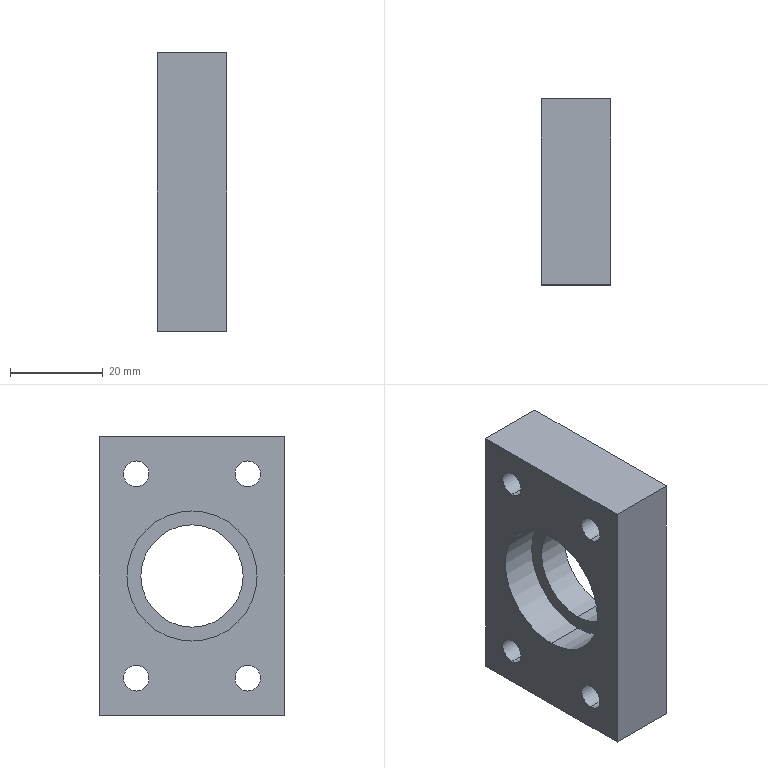Component | SolidWorks | ElectricalBoxAssembly2-1_BearingHousing-1 | 1 solid | 31 faces | box 15 x 40 x 60 mm | volume 26190 mm3 | cylinder 20 | plane 11 | commonest cylinder face diameters 9 x8 5.5 x8 22 x2 28 x2
build123d program:
from build123d import *

# Parameters (mm, degrees)
SKETCH1_W                                       = 60
SKETCH1_H                                       = 40
BOSS_EXTRUDE1_DEPTH                             = 7.5
SKETCH2_R                                       = 14
CUT_EXTRUDE1_DEPTH                              = 8
SKETCH6_R                                       = 11
CUT_EXTRUDE3_DEPTH                              = 37.932
M5_HEX_SOCKET_HEAD_CAP_SCREW_CBORE1_D           = 5.5
M5_HEX_SOCKET_HEAD_CAP_SCREW_CBORE1_CBORE_D     = 9
M5_HEX_SOCKET_HEAD_CAP_SCREW_CBORE1_CBORE_DEPTH = 5


with BuildPart() as part:
    # Sketch1 → Boss-Extrude1 (new, symmetric)
    with BuildSketch(Plane.XY):
        Rectangle(SKETCH1_W, SKETCH1_H)
    extrude(amount=BOSS_EXTRUDE1_DEPTH, both=True)

    # Sketch2 → Cut-Extrude1 (cut)
    with BuildSketch(Plane.XY.offset(7.5)):
        Circle(SKETCH2_R)
    extrude(amount=-CUT_EXTRUDE1_DEPTH, mode=Mode.SUBTRACT)

    # Sketch6 → Cut-Extrude3 (cut, through all)
    with BuildSketch(Plane.XY.offset(-0.5)):
        Circle(SKETCH6_R)
    extrude(amount=-CUT_EXTRUDE3_DEPTH, mode=Mode.SUBTRACT)

    # M5 Hex Socket Head Cap Screw CBORE1 (through all)
    with Locations(Plane(origin=(0, 0, -7.5), x_dir=(-1, 0, 0), z_dir=(0, 0, -1))):
        with Locations((-22, 12), (22, 12), (22, -12), (-22, -12)):
            CounterBoreHole(M5_HEX_SOCKET_HEAD_CAP_SCREW_CBORE1_D / 2, M5_HEX_SOCKET_HEAD_CAP_SCREW_CBORE1_CBORE_D / 2, M5_HEX_SOCKET_HEAD_CAP_SCREW_CBORE1_CBORE_DEPTH)


solid = part.part

# Placed as in the assembly
solid = solid.moved(Location((776.468, 214.666, 1676.399), (0, -90, 0)))
STEP:
#1=COLOUR_RGB('',0.7922,0.8196,0.9333);
#2=FILL_AREA_STYLE_COLOUR('',#1);
#3=FILL_AREA_STYLE('',(#2));
#4=SURFACE_STYLE_FILL_AREA(#3);
#5=SURFACE_SIDE_STYLE('',(#4));
#6=SURFACE_STYLE_USAGE(.BOTH.,#5);
#7=PRESENTATION_STYLE_ASSIGNMENT((#6));
#8=CARTESIAN_POINT('',(30.668,7.979,64.957));
#9=VERTEX_POINT('',#8);
#10=CARTESIAN_POINT('',(30.668,7.979,65.311));
#11=VERTEX_POINT('',#10);
#12=CARTESIAN_POINT('',(30.668,7.979,65.134));
#13=DIRECTION('',(1.,0.,0.));
#14=DIRECTION('',(0.,0.,1.));
#15=AXIS2_PLACEMENT_3D('',#12,#13,#14);
#16=CIRCLE('',#15,0.1772);
#17=EDGE_CURVE('',#9,#11,#16,.T.);
#18=ORIENTED_EDGE('',*,*,#17,.F.);
#19=CARTESIAN_POINT('',(30.865,7.979,64.957));
#20=VERTEX_POINT('',#19);
#21=CARTESIAN_POINT('',(30.865,7.979,64.957));
#22=DIRECTION('',(1.,0.,0.));
#23=VECTOR('',#22,39.37);
#24=LINE('',#21,#23);
#25=EDGE_CURVE('',#9,#20,#24,.T.);
#26=ORIENTED_EDGE('',*,*,#25,.T.);
#27=CARTESIAN_POINT('',(30.865,7.979,65.311));
#28=VERTEX_POINT('',#27);
#29=CARTESIAN_POINT('',(30.865,7.979,65.134));
#30=DIRECTION('',(1.,0.,0.));
#31=DIRECTION('',(0.,0.,1.));
#32=AXIS2_PLACEMENT_3D('',#29,#30,#31);
#33=CIRCLE('',#32,0.1772);
#34=EDGE_CURVE('',#20,#28,#33,.T.);
#35=ORIENTED_EDGE('',*,*,#34,.T.);
#36=CARTESIAN_POINT('',(30.865,7.979,65.311));
#37=DIRECTION('',(1.,0.,0.));
#38=VECTOR('',#37,39.37);
#39=LINE('',#36,#38);
#40=EDGE_CURVE('',#11,#28,#39,.T.);
#41=ORIENTED_EDGE('',*,*,#40,.F.);
#42=EDGE_LOOP('',(#18,#26,#35,#41));
#43=FACE_OUTER_BOUND('',#42,.T.);
#44=CARTESIAN_POINT('',(30.865,7.979,65.134));
#45=DIRECTION('',(1.,0.,0.));
#46=DIRECTION('',(0.,0.,1.));
#47=AXIS2_PLACEMENT_3D('',#44,#45,#46);
#48=CYLINDRICAL_SURFACE('',#47,0.1772);
#49=ADVANCED_FACE('',(#43),#48,.F.);
#50=CARTESIAN_POINT('',(30.274,7.979,65.026));
#51=VERTEX_POINT('',#50);
#52=CARTESIAN_POINT('',(30.274,7.979,65.242));
#53=VERTEX_POINT('',#52);
#54=CARTESIAN_POINT('',(30.274,7.979,65.134));
#55=DIRECTION('',(1.,0.,0.));
#56=DIRECTION('',(0.,0.,1.));
#57=AXIS2_PLACEMENT_3D('',#54,#55,#56);
#58=CIRCLE('',#57,0.1083);
#59=EDGE_CURVE('',#51,#53,#58,.T.);
#60=ORIENTED_EDGE('',*,*,#59,.F.);
#61=CARTESIAN_POINT('',(30.668,7.979,65.026));
#62=VERTEX_POINT('',#61);
#63=CARTESIAN_POINT('',(30.865,7.979,65.026));
#64=DIRECTION('',(1.,0.,0.));
#65=VECTOR('',#64,39.37);
#66=LINE('',#63,#65);
#67=EDGE_CURVE('',#51,#62,#66,.T.);
#68=ORIENTED_EDGE('',*,*,#67,.T.);
#69=CARTESIAN_POINT('',(30.668,7.979,65.242));
#70=VERTEX_POINT('',#69);
#71=CARTESIAN_POINT('',(30.668,7.979,65.134));
#72=DIRECTION('',(1.,0.,0.));
#73=DIRECTION('',(0.,0.,1.));
#74=AXIS2_PLACEMENT_3D('',#71,#72,#73);
#75=CIRCLE('',#74,0.1083);
#76=EDGE_CURVE('',#62,#70,#75,.T.);
#77=ORIENTED_EDGE('',*,*,#76,.T.);
#78=CARTESIAN_POINT('',(30.865,7.979,65.242));
#79=DIRECTION('',(1.,0.,0.));
#80=VECTOR('',#79,39.37);
#81=LINE('',#78,#80);
#82=EDGE_CURVE('',#53,#70,#81,.T.);
#83=ORIENTED_EDGE('',*,*,#82,.F.);
#84=EDGE_LOOP('',(#60,#68,#77,#83));
#85=FACE_OUTER_BOUND('',#84,.T.);
#86=CARTESIAN_POINT('',(30.865,7.979,65.134));
#87=DIRECTION('',(1.,0.,0.));
#88=DIRECTION('',(0.,0.,1.));
#89=AXIS2_PLACEMENT_3D('',#86,#87,#88);
#90=CYLINDRICAL_SURFACE('',#89,0.1083);
#91=ADVANCED_FACE('',(#85),#90,.F.);
#92=CARTESIAN_POINT('',(30.668,7.979,66.689));
#93=VERTEX_POINT('',#92);
#94=CARTESIAN_POINT('',(30.668,7.979,67.043));
#95=VERTEX_POINT('',#94);
#96=CARTESIAN_POINT('',(30.668,7.979,66.866));
#97=DIRECTION('',(1.,0.,0.));
#98=DIRECTION('',(0.,0.,1.));
#99=AXIS2_PLACEMENT_3D('',#96,#97,#98);
#100=CIRCLE('',#99,0.1772);
#101=EDGE_CURVE('',#93,#95,#100,.T.);
#102=ORIENTED_EDGE('',*,*,#101,.F.);
#103=CARTESIAN_POINT('',(30.865,7.979,66.689));
#104=VERTEX_POINT('',#103);
#105=CARTESIAN_POINT('',(30.865,7.979,66.689));
#106=DIRECTION('',(1.,0.,0.));
#107=VECTOR('',#106,39.37);
#108=LINE('',#105,#107);
#109=EDGE_CURVE('',#93,#104,#108,.T.);
#110=ORIENTED_EDGE('',*,*,#109,.T.);
#111=CARTESIAN_POINT('',(30.865,7.979,67.043));
#112=VERTEX_POINT('',#111);
#113=CARTESIAN_POINT('',(30.865,7.979,66.866));
#114=DIRECTION('',(1.,0.,0.));
#115=DIRECTION('',(0.,0.,1.));
#116=AXIS2_PLACEMENT_3D('',#113,#114,#115);
#117=CIRCLE('',#116,0.1772);
#118=EDGE_CURVE('',#104,#112,#117,.T.);
#119=ORIENTED_EDGE('',*,*,#118,.T.);
#120=CARTESIAN_POINT('',(30.865,7.979,67.043));
#121=DIRECTION('',(1.,0.,0.));
#122=VECTOR('',#121,39.37);
#123=LINE('',#120,#122);
#124=EDGE_CURVE('',#95,#112,#123,.T.);
#125=ORIENTED_EDGE('',*,*,#124,.F.);
#126=EDGE_LOOP('',(#102,#110,#119,#125));
#127=FACE_OUTER_BOUND('',#126,.T.);
#128=CARTESIAN_POINT('',(30.865,7.979,66.866));
#129=DIRECTION('',(1.,0.,0.));
#130=DIRECTION('',(0.,0.,1.));
#131=AXIS2_PLACEMENT_3D('',#128,#129,#130);
#132=CYLINDRICAL_SURFACE('',#131,0.1772);
#133=ADVANCED_FACE('',(#127),#132,.F.);
#134=CARTESIAN_POINT('',(30.274,7.979,66.758));
#135=VERTEX_POINT('',#134);
#136=CARTESIAN_POINT('',(30.274,7.979,66.974));
#137=VERTEX_POINT('',#136);
#138=CARTESIAN_POINT('',(30.274,7.979,66.866));
#139=DIRECTION('',(1.,0.,0.));
#140=DIRECTION('',(0.,0.,1.));
#141=AXIS2_PLACEMENT_3D('',#138,#139,#140);
#142=CIRCLE('',#141,0.1083);
#143=EDGE_CURVE('',#135,#137,#142,.T.);
#144=ORIENTED_EDGE('',*,*,#143,.F.);
#145=CARTESIAN_POINT('',(30.668,7.979,66.758));
#146=VERTEX_POINT('',#145);
#147=CARTESIAN_POINT('',(30.865,7.979,66.758));
#148=DIRECTION('',(1.,0.,0.));
#149=VECTOR('',#148,39.37);
#150=LINE('',#147,#149);
#151=EDGE_CURVE('',#135,#146,#150,.T.);
#152=ORIENTED_EDGE('',*,*,#151,.T.);
#153=CARTESIAN_POINT('',(30.668,7.979,66.974));
#154=VERTEX_POINT('',#153);
#155=CARTESIAN_POINT('',(30.668,7.979,66.866));
#156=DIRECTION('',(1.,0.,0.));
#157=DIRECTION('',(0.,0.,1.));
#158=AXIS2_PLACEMENT_3D('',#155,#156,#157);
#159=CIRCLE('',#158,0.1083);
#160=EDGE_CURVE('',#146,#154,#159,.T.);
#161=ORIENTED_EDGE('',*,*,#160,.T.);
#162=CARTESIAN_POINT('',(30.865,7.979,66.974));
#163=DIRECTION('',(1.,0.,0.));
#164=VECTOR('',#163,39.37);
#165=LINE('',#162,#164);
#166=EDGE_CURVE('',#137,#154,#165,.T.);
#167=ORIENTED_EDGE('',*,*,#166,.F.);
#168=EDGE_LOOP('',(#144,#152,#161,#167));
#169=FACE_OUTER_BOUND('',#168,.T.);
#170=CARTESIAN_POINT('',(30.865,7.979,66.866));
#171=DIRECTION('',(1.,0.,0.));
#172=DIRECTION('',(0.,0.,1.));
#173=AXIS2_PLACEMENT_3D('',#170,#171,#172);
#174=CYLINDRICAL_SURFACE('',#173,0.1083);
#175=ADVANCED_FACE('',(#169),#174,.F.);
#176=CARTESIAN_POINT('',(30.668,8.924,66.689));
#177=VERTEX_POINT('',#176);
#178=CARTESIAN_POINT('',(30.668,8.924,67.043));
#179=VERTEX_POINT('',#178);
#180=CARTESIAN_POINT('',(30.668,8.924,66.866));
#181=DIRECTION('',(1.,0.,0.));
#182=DIRECTION('',(0.,0.,1.));
#183=AXIS2_PLACEMENT_3D('',#180,#181,#182);
#184=CIRCLE('',#183,0.1772);
#185=EDGE_CURVE('',#177,#179,#184,.T.);
#186=ORIENTED_EDGE('',*,*,#185,.F.);
#187=CARTESIAN_POINT('',(30.865,8.924,66.689));
#188=VERTEX_POINT('',#187);
#189=CARTESIAN_POINT('',(30.865,8.924,66.689));
#190=DIRECTION('',(1.,0.,0.));
#191=VECTOR('',#190,39.37);
#192=LINE('',#189,#191);
#193=EDGE_CURVE('',#177,#188,#192,.T.);
#194=ORIENTED_EDGE('',*,*,#193,.T.);
#195=CARTESIAN_POINT('',(30.865,8.924,67.043));
#196=VERTEX_POINT('',#195);
#197=CARTESIAN_POINT('',(30.865,8.924,66.866));
#198=DIRECTION('',(1.,0.,0.));
#199=DIRECTION('',(0.,0.,1.));
#200=AXIS2_PLACEMENT_3D('',#197,#198,#199);
#201=CIRCLE('',#200,0.1772);
#202=EDGE_CURVE('',#188,#196,#201,.T.);
#203=ORIENTED_EDGE('',*,*,#202,.T.);
#204=CARTESIAN_POINT('',(30.865,8.924,67.043));
#205=DIRECTION('',(1.,0.,0.));
#206=VECTOR('',#205,39.37);
#207=LINE('',#204,#206);
#208=EDGE_CURVE('',#179,#196,#207,.T.);
#209=ORIENTED_EDGE('',*,*,#208,.F.);
#210=EDGE_LOOP('',(#186,#194,#203,#209));
#211=FACE_OUTER_BOUND('',#210,.T.);
#212=CARTESIAN_POINT('',(30.865,8.924,66.866));
#213=DIRECTION('',(1.,0.,0.));
#214=DIRECTION('',(0.,0.,1.));
#215=AXIS2_PLACEMENT_3D('',#212,#213,#214);
#216=CYLINDRICAL_SURFACE('',#215,0.1772);
#217=ADVANCED_FACE('',(#211),#216,.F.);
#218=CARTESIAN_POINT('',(30.274,8.924,66.758));
#219=VERTEX_POINT('',#218);
#220=CARTESIAN_POINT('',(30.274,8.924,66.974));
#221=VERTEX_POINT('',#220);
#222=CARTESIAN_POINT('',(30.274,8.924,66.866));
#223=DIRECTION('',(1.,0.,0.));
#224=DIRECTION('',(0.,0.,1.));
#225=AXIS2_PLACEMENT_3D('',#222,#223,#224);
#226=CIRCLE('',#225,0.1083);
#227=EDGE_CURVE('',#219,#221,#226,.T.);
#228=ORIENTED_EDGE('',*,*,#227,.F.);
#229=CARTESIAN_POINT('',(30.668,8.924,66.758));
#230=VERTEX_POINT('',#229);
#231=CARTESIAN_POINT('',(30.865,8.924,66.758));
#232=DIRECTION('',(1.,0.,0.));
#233=VECTOR('',#232,39.37);
#234=LINE('',#231,#233);
#235=EDGE_CURVE('',#219,#230,#234,.T.);
#236=ORIENTED_EDGE('',*,*,#235,.T.);
#237=CARTESIAN_POINT('',(30.668,8.924,66.974));
#238=VERTEX_POINT('',#237);
#239=CARTESIAN_POINT('',(30.668,8.924,66.866));
#240=DIRECTION('',(1.,0.,0.));
#241=DIRECTION('',(0.,0.,1.));
#242=AXIS2_PLACEMENT_3D('',#239,#240,#241);
#243=CIRCLE('',#242,0.1083);
#244=EDGE_CURVE('',#230,#238,#243,.T.);
#245=ORIENTED_EDGE('',*,*,#244,.T.);
#246=CARTESIAN_POINT('',(30.865,8.924,66.974));
#247=DIRECTION('',(1.,0.,0.));
#248=VECTOR('',#247,39.37);
#249=LINE('',#246,#248);
#250=EDGE_CURVE('',#221,#238,#249,.T.);
#251=ORIENTED_EDGE('',*,*,#250,.F.);
#252=EDGE_LOOP('',(#228,#236,#245,#251));
#253=FACE_OUTER_BOUND('',#252,.T.);
#254=CARTESIAN_POINT('',(30.865,8.924,66.866));
#255=DIRECTION('',(1.,0.,0.));
#256=DIRECTION('',(0.,0.,1.));
#257=AXIS2_PLACEMENT_3D('',#254,#255,#256);
#258=CYLINDRICAL_SURFACE('',#257,0.1083);
#259=ADVANCED_FACE('',(#253),#258,.F.);
#260=CARTESIAN_POINT('',(30.668,8.924,64.957));
#261=VERTEX_POINT('',#260);
#262=CARTESIAN_POINT('',(30.668,8.924,65.311));
#263=VERTEX_POINT('',#262);
#264=CARTESIAN_POINT('',(30.668,8.924,65.134));
#265=DIRECTION('',(1.,0.,0.));
#266=DIRECTION('',(0.,0.,1.));
#267=AXIS2_PLACEMENT_3D('',#264,#265,#266);
#268=CIRCLE('',#267,0.1772);
#269=EDGE_CURVE('',#261,#263,#268,.T.);
#270=ORIENTED_EDGE('',*,*,#269,.F.);
#271=CARTESIAN_POINT('',(30.865,8.924,64.957));
#272=VERTEX_POINT('',#271);
#273=CARTESIAN_POINT('',(30.865,8.924,64.957));
#274=DIRECTION('',(1.,0.,0.));
#275=VECTOR('',#274,39.37);
#276=LINE('',#273,#275);
#277=EDGE_CURVE('',#261,#272,#276,.T.);
#278=ORIENTED_EDGE('',*,*,#277,.T.);
#279=CARTESIAN_POINT('',(30.865,8.924,65.311));
#280=VERTEX_POINT('',#279);
#281=CARTESIAN_POINT('',(30.865,8.924,65.134));
#282=DIRECTION('',(1.,0.,0.));
#283=DIRECTION('',(0.,0.,1.));
#284=AXIS2_PLACEMENT_3D('',#281,#282,#283);
#285=CIRCLE('',#284,0.1772);
#286=EDGE_CURVE('',#272,#280,#285,.T.);
#287=ORIENTED_EDGE('',*,*,#286,.T.);
#288=CARTESIAN_POINT('',(30.865,8.924,65.311));
#289=DIRECTION('',(1.,0.,0.));
#290=VECTOR('',#289,39.37);
#291=LINE('',#288,#290);
#292=EDGE_CURVE('',#263,#280,#291,.T.);
#293=ORIENTED_EDGE('',*,*,#292,.F.);
#294=EDGE_LOOP('',(#270,#278,#287,#293));
#295=FACE_OUTER_BOUND('',#294,.T.);
#296=CARTESIAN_POINT('',(30.865,8.924,65.134));
#297=DIRECTION('',(1.,0.,0.));
#298=DIRECTION('',(0.,0.,1.));
#299=AXIS2_PLACEMENT_3D('',#296,#297,#298);
#300=CYLINDRICAL_SURFACE('',#299,0.1772);
#301=ADVANCED_FACE('',(#295),#300,.F.);
#302=CARTESIAN_POINT('',(30.274,8.924,65.026));
#303=VERTEX_POINT('',#302);
#304=CARTESIAN_POINT('',(30.274,8.924,65.242));
#305=VERTEX_POINT('',#304);
#306=CARTESIAN_POINT('',(30.274,8.924,65.134));
#307=DIRECTION('',(1.,0.,0.));
#308=DIRECTION('',(0.,0.,1.));
#309=AXIS2_PLACEMENT_3D('',#306,#307,#308);
#310=CIRCLE('',#309,0.1083);
#311=EDGE_CURVE('',#303,#305,#310,.T.);
#312=ORIENTED_EDGE('',*,*,#311,.F.);
#313=CARTESIAN_POINT('',(30.668,8.924,65.026));
#314=VERTEX_POINT('',#313);
#315=CARTESIAN_POINT('',(30.865,8.924,65.026));
#316=DIRECTION('',(1.,0.,0.));
#317=VECTOR('',#316,39.37);
#318=LINE('',#315,#317);
#319=EDGE_CURVE('',#303,#314,#318,.T.);
#320=ORIENTED_EDGE('',*,*,#319,.T.);
#321=CARTESIAN_POINT('',(30.668,8.924,65.242));
#322=VERTEX_POINT('',#321);
#323=CARTESIAN_POINT('',(30.668,8.924,65.134));
#324=DIRECTION('',(1.,0.,0.));
#325=DIRECTION('',(0.,0.,1.));
#326=AXIS2_PLACEMENT_3D('',#323,#324,#325);
#327=CIRCLE('',#326,0.1083);
#328=EDGE_CURVE('',#314,#322,#327,.T.);
#329=ORIENTED_EDGE('',*,*,#328,.T.);
#330=CARTESIAN_POINT('',(30.865,8.924,65.242));
#331=DIRECTION('',(1.,0.,0.));
#332=VECTOR('',#331,39.37);
#333=LINE('',#330,#332);
#334=EDGE_CURVE('',#305,#322,#333,.T.);
#335=ORIENTED_EDGE('',*,*,#334,.F.);
#336=EDGE_LOOP('',(#312,#320,#329,#335));
#337=FACE_OUTER_BOUND('',#336,.T.);
#338=CARTESIAN_POINT('',(30.865,8.924,65.134));
#339=DIRECTION('',(1.,0.,0.));
#340=DIRECTION('',(0.,0.,1.));
#341=AXIS2_PLACEMENT_3D('',#338,#339,#340);
#342=CYLINDRICAL_SURFACE('',#341,0.1083);
#343=ADVANCED_FACE('',(#337),#342,.F.);
#344=CARTESIAN_POINT('',(30.865,8.451,66.433));
#345=VERTEX_POINT('',#344);
#346=CARTESIAN_POINT('',(30.865,8.451,65.567));
#347=VERTEX_POINT('',#346);
#348=CARTESIAN_POINT('',(30.865,8.451,66.));
#349=DIRECTION('',(-1.,-0.,-0.));
#350=DIRECTION('',(0.,0.,-1.));
#351=AXIS2_PLACEMENT_3D('',#348,#349,#350);
#352=CIRCLE('',#351,0.4331);
#353=EDGE_CURVE('',#345,#347,#352,.T.);
#354=ORIENTED_EDGE('',*,*,#353,.F.);
#355=CARTESIAN_POINT('',(30.589,8.451,66.433));
#356=VERTEX_POINT('',#355);
#357=CARTESIAN_POINT('',(30.865,8.451,66.433));
#358=DIRECTION('',(-1.,-0.,-0.));
#359=VECTOR('',#358,39.37);
#360=LINE('',#357,#359);
#361=EDGE_CURVE('',#345,#356,#360,.T.);
#362=ORIENTED_EDGE('',*,*,#361,.T.);
#363=CARTESIAN_POINT('',(30.589,8.451,65.567));
#364=VERTEX_POINT('',#363);
#365=CARTESIAN_POINT('',(30.589,8.451,66.));
#366=DIRECTION('',(-1.,-0.,-0.));
#367=DIRECTION('',(0.,0.,-1.));
#368=AXIS2_PLACEMENT_3D('',#365,#366,#367);
#369=CIRCLE('',#368,0.4331);
#370=EDGE_CURVE('',#356,#364,#369,.T.);
#371=ORIENTED_EDGE('',*,*,#370,.T.);
#372=CARTESIAN_POINT('',(30.865,8.451,65.567));
#373=DIRECTION('',(-1.,-0.,-0.));
#374=VECTOR('',#373,39.37);
#375=LINE('',#372,#374);
#376=EDGE_CURVE('',#347,#364,#375,.T.);
#377=ORIENTED_EDGE('',*,*,#376,.F.);
#378=EDGE_LOOP('',(#354,#362,#371,#377));
#379=FACE_OUTER_BOUND('',#378,.T.);
#380=CARTESIAN_POINT('',(30.865,8.451,66.));
#381=DIRECTION('',(-1.,-0.,-0.));
#382=DIRECTION('',(0.,0.,-1.));
#383=AXIS2_PLACEMENT_3D('',#380,#381,#382);
#384=CYLINDRICAL_SURFACE('',#383,0.4331);
#385=ADVANCED_FACE('',(#379),#384,.F.);
#386=CARTESIAN_POINT('',(30.589,8.451,66.551));
#387=VERTEX_POINT('',#386);
#388=CARTESIAN_POINT('',(30.589,8.451,65.449));
#389=VERTEX_POINT('',#388);
#390=CARTESIAN_POINT('',(30.589,8.451,66.));
#391=DIRECTION('',(-1.,-0.,-0.));
#392=DIRECTION('',(0.,0.,-1.));
#393=AXIS2_PLACEMENT_3D('',#390,#391,#392);
#394=CIRCLE('',#393,0.5512);
#395=EDGE_CURVE('',#387,#389,#394,.T.);
#396=ORIENTED_EDGE('',*,*,#395,.F.);
#397=CARTESIAN_POINT('',(30.274,8.451,66.551));
#398=VERTEX_POINT('',#397);
#399=CARTESIAN_POINT('',(30.589,8.451,66.551));
#400=DIRECTION('',(-1.,-0.,-0.));
#401=VECTOR('',#400,39.37);
#402=LINE('',#399,#401);
#403=EDGE_CURVE('',#387,#398,#402,.T.);
#404=ORIENTED_EDGE('',*,*,#403,.T.);
#405=CARTESIAN_POINT('',(30.274,8.451,65.449));
#406=VERTEX_POINT('',#405);
#407=CARTESIAN_POINT('',(30.274,8.451,66.));
#408=DIRECTION('',(-1.,-0.,-0.));
#409=DIRECTION('',(0.,0.,-1.));
#410=AXIS2_PLACEMENT_3D('',#407,#408,#409);
#411=CIRCLE('',#410,0.5512);
#412=EDGE_CURVE('',#398,#406,#411,.T.);
#413=ORIENTED_EDGE('',*,*,#412,.T.);
#414=CARTESIAN_POINT('',(30.589,8.451,65.449));
#415=DIRECTION('',(-1.,-0.,-0.));
#416=VECTOR('',#415,39.37);
#417=LINE('',#414,#416);
#418=EDGE_CURVE('',#389,#406,#417,.T.);
#419=ORIENTED_EDGE('',*,*,#418,.F.);
#420=EDGE_LOOP('',(#396,#404,#413,#419));
#421=FACE_OUTER_BOUND('',#420,.T.);
#422=CARTESIAN_POINT('',(30.589,8.451,66.));
#423=DIRECTION('',(-1.,-0.,-0.));
#424=DIRECTION('',(0.,0.,-1.));
#425=AXIS2_PLACEMENT_3D('',#422,#423,#424);
#426=CYLINDRICAL_SURFACE('',#425,0.5512);
#427=ADVANCED_FACE('',(#421),#426,.F.);
#428=CARTESIAN_POINT('',(30.865,9.239,64.819));
#429=VERTEX_POINT('',#428);
#430=CARTESIAN_POINT('',(30.865,7.664,64.819));
#431=VERTEX_POINT('',#430);
#432=CARTESIAN_POINT('',(30.865,7.664,64.819));
#433=DIRECTION('',(-0.,-1.,-0.));
#434=VECTOR('',#433,39.37);
#435=LINE('',#432,#434);
#436=EDGE_CURVE('',#429,#431,#435,.T.);
#437=ORIENTED_EDGE('',*,*,#436,.T.);
#438=CARTESIAN_POINT('',(30.274,7.664,64.819));
#439=VERTEX_POINT('',#438);
#440=CARTESIAN_POINT('',(30.274,7.664,64.819));
#441=DIRECTION('',(1.,0.,0.));
#442=VECTOR('',#441,39.37);
#443=LINE('',#440,#442);
#444=EDGE_CURVE('',#439,#431,#443,.T.);
#445=ORIENTED_EDGE('',*,*,#444,.F.);
#446=CARTESIAN_POINT('',(30.274,9.239,64.819));
#447=VERTEX_POINT('',#446);
#448=CARTESIAN_POINT('',(30.274,7.664,64.819));
#449=DIRECTION('',(-0.,-1.,-0.));
#450=VECTOR('',#449,39.37);
#451=LINE('',#448,#450);
#452=EDGE_CURVE('',#447,#439,#451,.T.);
#453=ORIENTED_EDGE('',*,*,#452,.F.);
#454=CARTESIAN_POINT('',(30.274,9.239,64.819));
#455=DIRECTION('',(1.,0.,0.));
#456=VECTOR('',#455,39.37);
#457=LINE('',#454,#456);
#458=EDGE_CURVE('',#447,#429,#457,.T.);
#459=ORIENTED_EDGE('',*,*,#458,.T.);
#460=EDGE_LOOP('',(#437,#445,#453,#459));
#461=FACE_OUTER_BOUND('',#460,.T.);
#462=CARTESIAN_POINT('',(30.274,7.664,64.819));
#463=DIRECTION('',(-0.,0.,1.));
#464=DIRECTION('',(-1.,-0.,-0.));
#465=AXIS2_PLACEMENT_3D('',#462,#463,#464);
#466=PLANE('',#465);
#467=ADVANCED_FACE('',(#461),#466,.F.);
#468=CARTESIAN_POINT('',(30.865,7.664,67.181));
#469=VERTEX_POINT('',#468);
#470=CARTESIAN_POINT('',(30.865,7.664,67.181));
#471=DIRECTION('',(-0.,0.,1.));
#472=VECTOR('',#471,39.37);
#473=LINE('',#470,#472);
#474=EDGE_CURVE('',#431,#469,#473,.T.);
#475=ORIENTED_EDGE('',*,*,#474,.T.);
#476=CARTESIAN_POINT('',(30.274,7.664,67.181));
#477=VERTEX_POINT('',#476);
#478=CARTESIAN_POINT('',(30.274,7.664,67.181));
#479=DIRECTION('',(1.,0.,0.));
#480=VECTOR('',#479,39.37);
#481=LINE('',#478,#480);
#482=EDGE_CURVE('',#477,#469,#481,.T.);
#483=ORIENTED_EDGE('',*,*,#482,.F.);
#484=CARTESIAN_POINT('',(30.274,7.664,67.181));
#485=DIRECTION('',(-0.,0.,1.));
#486=VECTOR('',#485,39.37);
#487=LINE('',#484,#486);
#488=EDGE_CURVE('',#439,#477,#487,.T.);
#489=ORIENTED_EDGE('',*,*,#488,.F.);
#490=ORIENTED_EDGE('',*,*,#444,.T.);
#491=EDGE_LOOP('',(#475,#483,#489,#490));
#492=FACE_OUTER_BOUND('',#491,.T.);
#493=CARTESIAN_POINT('',(30.274,7.664,67.181));
#494=DIRECTION('',(-0.,1.,0.));
#495=DIRECTION('',(1.,0.,0.));
#496=AXIS2_PLACEMENT_3D('',#493,#494,#495);
#497=PLANE('',#496);
#498=ADVANCED_FACE('',(#492),#497,.F.);
#499=CARTESIAN_POINT('',(30.865,9.239,67.181));
#500=VERTEX_POINT('',#499);
#501=CARTESIAN_POINT('',(30.865,7.664,67.181));
#502=DIRECTION('',(-0.,1.,0.));
#503=VECTOR('',#502,39.37);
#504=LINE('',#501,#503);
#505=EDGE_CURVE('',#469,#500,#504,.T.);
#506=ORIENTED_EDGE('',*,*,#505,.T.);
#507=CARTESIAN_POINT('',(30.274,9.239,67.181));
#508=VERTEX_POINT('',#507);
#509=CARTESIAN_POINT('',(30.274,9.239,67.181));
#510=DIRECTION('',(1.,0.,0.));
#511=VECTOR('',#510,39.37);
#512=LINE('',#509,#511);
#513=EDGE_CURVE('',#508,#500,#512,.T.);
#514=ORIENTED_EDGE('',*,*,#513,.F.);
#515=CARTESIAN_POINT('',(30.274,7.664,67.181));
#516=DIRECTION('',(-0.,1.,0.));
#517=VECTOR('',#516,39.37);
#518=LINE('',#515,#517);
#519=EDGE_CURVE('',#477,#508,#518,.T.);
#520=ORIENTED_EDGE('',*,*,#519,.F.);
#521=ORIENTED_EDGE('',*,*,#482,.T.);
#522=EDGE_LOOP('',(#506,#514,#520,#521));
#523=FACE_OUTER_BOUND('',#522,.T.);
#524=CARTESIAN_POINT('',(30.274,7.664,67.181));
#525=DIRECTION('',(0.,0.,-1.));
#526=DIRECTION('',(0.,-1.,-0.));
#527=AXIS2_PLACEMENT_3D('',#524,#525,#526);
#528=PLANE('',#527);
#529=ADVANCED_FACE('',(#523),#528,.F.);
#530=CARTESIAN_POINT('',(30.865,9.239,67.181));
#531=DIRECTION('',(0.,-0.,-1.));
#532=VECTOR('',#531,39.37);
#533=LINE('',#530,#532);
#534=EDGE_CURVE('',#500,#429,#533,.T.);
#535=ORIENTED_EDGE('',*,*,#534,.T.);
#536=ORIENTED_EDGE('',*,*,#458,.F.);
#537=CARTESIAN_POINT('',(30.274,9.239,67.181));
#538=DIRECTION('',(0.,-0.,-1.));
#539=VECTOR('',#538,39.37);
#540=LINE('',#537,#539);
#541=EDGE_CURVE('',#508,#447,#540,.T.);
#542=ORIENTED_EDGE('',*,*,#541,.F.);
#543=ORIENTED_EDGE('',*,*,#513,.T.);
#544=EDGE_LOOP('',(#535,#536,#542,#543));
#545=FACE_OUTER_BOUND('',#544,.T.);
#546=CARTESIAN_POINT('',(30.274,9.239,67.181));
#547=DIRECTION('',(0.,-1.,-0.));
#548=DIRECTION('',(-1.,-0.,-0.));
#549=AXIS2_PLACEMENT_3D('',#546,#547,#548);
#550=PLANE('',#549);
#551=ADVANCED_FACE('',(#545),#550,.F.);
#552=CARTESIAN_POINT('',(30.274,7.979,65.134));
#553=DIRECTION('',(1.,0.,0.));
#554=DIRECTION('',(0.,0.,1.));
#555=AXIS2_PLACEMENT_3D('',#552,#553,#554);
#556=CIRCLE('',#555,0.1083);
#557=EDGE_CURVE('',#53,#51,#556,.T.);
#558=ORIENTED_EDGE('',*,*,#557,.T.);
#559=ORIENTED_EDGE('',*,*,#59,.T.);
#560=EDGE_LOOP('',(#558,#559));
#561=FACE_BOUND('',#560,.T.);
#562=CARTESIAN_POINT('',(30.274,7.979,66.866));
#563=DIRECTION('',(1.,0.,0.));
#564=DIRECTION('',(0.,0.,1.));
#565=AXIS2_PLACEMENT_3D('',#562,#563,#564);
#566=CIRCLE('',#565,0.1083);
#567=EDGE_CURVE('',#137,#135,#566,.T.);
#568=ORIENTED_EDGE('',*,*,#567,.T.);
#569=ORIENTED_EDGE('',*,*,#143,.T.);
#570=EDGE_LOOP('',(#568,#569));
#571=FACE_BOUND('',#570,.T.);
#572=CARTESIAN_POINT('',(30.274,8.924,66.866));
#573=DIRECTION('',(1.,0.,0.));
#574=DIRECTION('',(0.,0.,1.));
#575=AXIS2_PLACEMENT_3D('',#572,#573,#574);
#576=CIRCLE('',#575,0.1083);
#577=EDGE_CURVE('',#221,#219,#576,.T.);
#578=ORIENTED_EDGE('',*,*,#577,.T.);
#579=ORIENTED_EDGE('',*,*,#227,.T.);
#580=EDGE_LOOP('',(#578,#579));
#581=FACE_BOUND('',#580,.T.);
#582=CARTESIAN_POINT('',(30.274,8.924,65.134));
#583=DIRECTION('',(1.,0.,0.));
#584=DIRECTION('',(0.,0.,1.));
#585=AXIS2_PLACEMENT_3D('',#582,#583,#584);
#586=CIRCLE('',#585,0.1083);
#587=EDGE_CURVE('',#305,#303,#586,.T.);
#588=ORIENTED_EDGE('',*,*,#587,.T.);
#589=ORIENTED_EDGE('',*,*,#311,.T.);
#590=EDGE_LOOP('',(#588,#589));
#591=FACE_BOUND('',#590,.T.);
#592=CARTESIAN_POINT('',(30.274,8.451,66.));
#593=DIRECTION('',(-1.,-0.,-0.));
#594=DIRECTION('',(0.,0.,-1.));
#595=AXIS2_PLACEMENT_3D('',#592,#593,#594);
#596=CIRCLE('',#595,0.5512);
#597=EDGE_CURVE('',#406,#398,#596,.T.);
#598=ORIENTED_EDGE('',*,*,#597,.F.);
#599=ORIENTED_EDGE('',*,*,#412,.F.);
#600=EDGE_LOOP('',(#598,#599));
#601=FACE_BOUND('',#600,.T.);
#602=ORIENTED_EDGE('',*,*,#452,.T.);
#603=ORIENTED_EDGE('',*,*,#488,.T.);
#604=ORIENTED_EDGE('',*,*,#519,.T.);
#605=ORIENTED_EDGE('',*,*,#541,.T.);
#606=EDGE_LOOP('',(#602,#603,#604,#605));
#607=FACE_OUTER_BOUND('',#606,.T.);
#608=CARTESIAN_POINT('',(30.274,8.451,66.));
#609=DIRECTION('',(-1.,-0.,-0.));
#610=DIRECTION('',(0.,-0.,-1.));
#611=AXIS2_PLACEMENT_3D('',#608,#609,#610);
#612=PLANE('',#611);
#613=ADVANCED_FACE('',(#561,#571,#581,#591,#601,#607),#612,.T.);
#614=CARTESIAN_POINT('',(30.865,7.979,65.134));
#615=DIRECTION('',(1.,0.,0.));
#616=DIRECTION('',(0.,0.,1.));
#617=AXIS2_PLACEMENT_3D('',#614,#615,#616);
#618=CIRCLE('',#617,0.1772);
#619=EDGE_CURVE('',#28,#20,#618,.T.);
#620=ORIENTED_EDGE('',*,*,#619,.F.);
#621=ORIENTED_EDGE('',*,*,#34,.F.);
#622=EDGE_LOOP('',(#620,#621));
#623=FACE_BOUND('',#622,.T.);
#624=CARTESIAN_POINT('',(30.865,7.979,66.866));
#625=DIRECTION('',(1.,0.,0.));
#626=DIRECTION('',(0.,0.,1.));
#627=AXIS2_PLACEMENT_3D('',#624,#625,#626);
#628=CIRCLE('',#627,0.1772);
#629=EDGE_CURVE('',#112,#104,#628,.T.);
#630=ORIENTED_EDGE('',*,*,#629,.F.);
#631=ORIENTED_EDGE('',*,*,#118,.F.);
#632=EDGE_LOOP('',(#630,#631));
#633=FACE_BOUND('',#632,.T.);
#634=CARTESIAN_POINT('',(30.865,8.924,66.866));
#635=DIRECTION('',(1.,0.,0.));
#636=DIRECTION('',(0.,0.,1.));
#637=AXIS2_PLACEMENT_3D('',#634,#635,#636);
#638=CIRCLE('',#637,0.1772);
#639=EDGE_CURVE('',#196,#188,#638,.T.);
#640=ORIENTED_EDGE('',*,*,#639,.F.);
#641=ORIENTED_EDGE('',*,*,#202,.F.);
#642=EDGE_LOOP('',(#640,#641));
#643=FACE_BOUND('',#642,.T.);
#644=CARTESIAN_POINT('',(30.865,8.924,65.134));
#645=DIRECTION('',(1.,0.,0.));
#646=DIRECTION('',(0.,0.,1.));
#647=AXIS2_PLACEMENT_3D('',#644,#645,#646);
#648=CIRCLE('',#647,0.1772);
#649=EDGE_CURVE('',#280,#272,#648,.T.);
#650=ORIENTED_EDGE('',*,*,#649,.F.);
#651=ORIENTED_EDGE('',*,*,#286,.F.);
#652=EDGE_LOOP('',(#650,#651));
#653=FACE_BOUND('',#652,.T.);
#654=CARTESIAN_POINT('',(30.865,8.451,66.));
#655=DIRECTION('',(-1.,-0.,-0.));
#656=DIRECTION('',(0.,0.,-1.));
#657=AXIS2_PLACEMENT_3D('',#654,#655,#656);
#658=CIRCLE('',#657,0.4331);
#659=EDGE_CURVE('',#347,#345,#658,.T.);
#660=ORIENTED_EDGE('',*,*,#659,.T.);
#661=ORIENTED_EDGE('',*,*,#353,.T.);
#662=EDGE_LOOP('',(#660,#661));
#663=FACE_BOUND('',#662,.T.);
#664=ORIENTED_EDGE('',*,*,#436,.F.);
#665=ORIENTED_EDGE('',*,*,#534,.F.);
#666=ORIENTED_EDGE('',*,*,#505,.F.);
#667=ORIENTED_EDGE('',*,*,#474,.F.);
#668=EDGE_LOOP('',(#664,#665,#666,#667));
#669=FACE_OUTER_BOUND('',#668,.T.);
#670=CARTESIAN_POINT('',(30.865,8.451,66.));
#671=DIRECTION('',(-1.,-0.,-0.));
#672=DIRECTION('',(0.,-0.,-1.));
#673=AXIS2_PLACEMENT_3D('',#670,#671,#672);
#674=PLANE('',#673);
#675=ADVANCED_FACE('',(#623,#633,#643,#653,#663,#669),#674,.F.);
#676=ORIENTED_EDGE('',*,*,#403,.F.);
#677=CARTESIAN_POINT('',(30.589,8.451,66.));
#678=DIRECTION('',(-1.,-0.,-0.));
#679=DIRECTION('',(0.,0.,-1.));
#680=AXIS2_PLACEMENT_3D('',#677,#678,#679);
#681=CIRCLE('',#680,0.5512);
#682=EDGE_CURVE('',#389,#387,#681,.T.);
#683=ORIENTED_EDGE('',*,*,#682,.F.);
#684=ORIENTED_EDGE('',*,*,#418,.T.);
#685=ORIENTED_EDGE('',*,*,#597,.T.);
#686=EDGE_LOOP('',(#676,#683,#684,#685));
#687=FACE_OUTER_BOUND('',#686,.T.);
#688=CARTESIAN_POINT('',(30.589,8.451,66.));
#689=DIRECTION('',(-1.,-0.,-0.));
#690=DIRECTION('',(0.,0.,-1.));
#691=AXIS2_PLACEMENT_3D('',#688,#689,#690);
#692=CYLINDRICAL_SURFACE('',#691,0.5512);
#693=ADVANCED_FACE('',(#687),#692,.F.);
#694=CARTESIAN_POINT('',(30.589,8.451,66.));
#695=DIRECTION('',(-1.,-0.,-0.));
#696=DIRECTION('',(0.,0.,-1.));
#697=AXIS2_PLACEMENT_3D('',#694,#695,#696);
#698=CIRCLE('',#697,0.4331);
#699=EDGE_CURVE('',#364,#356,#698,.T.);
#700=ORIENTED_EDGE('',*,*,#699,.F.);
#701=ORIENTED_EDGE('',*,*,#370,.F.);
#702=EDGE_LOOP('',(#700,#701));
#703=FACE_BOUND('',#702,.T.);
#704=ORIENTED_EDGE('',*,*,#682,.T.);
#705=ORIENTED_EDGE('',*,*,#395,.T.);
#706=EDGE_LOOP('',(#704,#705));
#707=FACE_OUTER_BOUND('',#706,.T.);
#708=CARTESIAN_POINT('',(30.589,8.451,66.));
#709=DIRECTION('',(-1.,-0.,-0.));
#710=DIRECTION('',(0.,-0.,-1.));
#711=AXIS2_PLACEMENT_3D('',#708,#709,#710);
#712=PLANE('',#711);
#713=ADVANCED_FACE('',(#703,#707),#712,.T.);
#714=ORIENTED_EDGE('',*,*,#361,.F.);
#715=ORIENTED_EDGE('',*,*,#659,.F.);
#716=ORIENTED_EDGE('',*,*,#376,.T.);
#717=ORIENTED_EDGE('',*,*,#699,.T.);
#718=EDGE_LOOP('',(#714,#715,#716,#717));
#719=FACE_OUTER_BOUND('',#718,.T.);
#720=CARTESIAN_POINT('',(30.865,8.451,66.));
#721=DIRECTION('',(-1.,-0.,-0.));
#722=DIRECTION('',(0.,0.,-1.));
#723=AXIS2_PLACEMENT_3D('',#720,#721,#722);
#724=CYLINDRICAL_SURFACE('',#723,0.4331);
#725=ADVANCED_FACE('',(#719),#724,.F.);
#726=ORIENTED_EDGE('',*,*,#319,.F.);
#727=ORIENTED_EDGE('',*,*,#587,.F.);
#728=ORIENTED_EDGE('',*,*,#334,.T.);
#729=CARTESIAN_POINT('',(30.668,8.924,65.134));
#730=DIRECTION('',(1.,0.,0.));
#731=DIRECTION('',(0.,0.,1.));
#732=AXIS2_PLACEMENT_3D('',#729,#730,#731);
#733=CIRCLE('',#732,0.1083);
#734=EDGE_CURVE('',#322,#314,#733,.T.);
#735=ORIENTED_EDGE('',*,*,#734,.T.);
#736=EDGE_LOOP('',(#726,#727,#728,#735));
#737=FACE_OUTER_BOUND('',#736,.T.);
#738=CARTESIAN_POINT('',(30.865,8.924,65.134));
#739=DIRECTION('',(1.,0.,0.));
#740=DIRECTION('',(0.,0.,1.));
#741=AXIS2_PLACEMENT_3D('',#738,#739,#740);
#742=CYLINDRICAL_SURFACE('',#741,0.1083);
#743=ADVANCED_FACE('',(#737),#742,.F.);
#744=ORIENTED_EDGE('',*,*,#734,.F.);
#745=ORIENTED_EDGE('',*,*,#328,.F.);
#746=EDGE_LOOP('',(#744,#745));
#747=FACE_BOUND('',#746,.T.);
#748=CARTESIAN_POINT('',(30.668,8.924,65.134));
#749=DIRECTION('',(1.,0.,0.));
#750=DIRECTION('',(0.,0.,1.));
#751=AXIS2_PLACEMENT_3D('',#748,#749,#750);
#752=CIRCLE('',#751,0.1772);
#753=EDGE_CURVE('',#263,#261,#752,.T.);
#754=ORIENTED_EDGE('',*,*,#753,.T.);
#755=ORIENTED_EDGE('',*,*,#269,.T.);
#756=EDGE_LOOP('',(#754,#755));
#757=FACE_OUTER_BOUND('',#756,.T.);
#758=CARTESIAN_POINT('',(30.668,8.924,65.026));
#759=DIRECTION('',(-1.,-0.,-0.));
#760=DIRECTION('',(0.,-0.,-1.));
#761=AXIS2_PLACEMENT_3D('',#758,#759,#760);
#762=PLANE('',#761);
#763=ADVANCED_FACE('',(#747,#757),#762,.F.);
#764=ORIENTED_EDGE('',*,*,#277,.F.);
#765=ORIENTED_EDGE('',*,*,#753,.F.);
#766=ORIENTED_EDGE('',*,*,#292,.T.);
#767=ORIENTED_EDGE('',*,*,#649,.T.);
#768=EDGE_LOOP('',(#764,#765,#766,#767));
#769=FACE_OUTER_BOUND('',#768,.T.);
#770=CARTESIAN_POINT('',(30.865,8.924,65.134));
#771=DIRECTION('',(1.,0.,0.));
#772=DIRECTION('',(0.,0.,1.));
#773=AXIS2_PLACEMENT_3D('',#770,#771,#772);
#774=CYLINDRICAL_SURFACE('',#773,0.1772);
#775=ADVANCED_FACE('',(#769),#774,.F.);
#776=ORIENTED_EDGE('',*,*,#235,.F.);
#777=ORIENTED_EDGE('',*,*,#577,.F.);
#778=ORIENTED_EDGE('',*,*,#250,.T.);
#779=CARTESIAN_POINT('',(30.668,8.924,66.866));
#780=DIRECTION('',(1.,0.,0.));
#781=DIRECTION('',(0.,0.,1.));
#782=AXIS2_PLACEMENT_3D('',#779,#780,#781);
#783=CIRCLE('',#782,0.1083);
#784=EDGE_CURVE('',#238,#230,#783,.T.);
#785=ORIENTED_EDGE('',*,*,#784,.T.);
#786=EDGE_LOOP('',(#776,#777,#778,#785));
#787=FACE_OUTER_BOUND('',#786,.T.);
#788=CARTESIAN_POINT('',(30.865,8.924,66.866));
#789=DIRECTION('',(1.,0.,0.));
#790=DIRECTION('',(0.,0.,1.));
#791=AXIS2_PLACEMENT_3D('',#788,#789,#790);
#792=CYLINDRICAL_SURFACE('',#791,0.1083);
#793=ADVANCED_FACE('',(#787),#792,.F.);
#794=ORIENTED_EDGE('',*,*,#784,.F.);
#795=ORIENTED_EDGE('',*,*,#244,.F.);
#796=EDGE_LOOP('',(#794,#795));
#797=FACE_BOUND('',#796,.T.);
#798=CARTESIAN_POINT('',(30.668,8.924,66.866));
#799=DIRECTION('',(1.,0.,0.));
#800=DIRECTION('',(0.,0.,1.));
#801=AXIS2_PLACEMENT_3D('',#798,#799,#800);
#802=CIRCLE('',#801,0.1772);
#803=EDGE_CURVE('',#179,#177,#802,.T.);
#804=ORIENTED_EDGE('',*,*,#803,.T.);
#805=ORIENTED_EDGE('',*,*,#185,.T.);
#806=EDGE_LOOP('',(#804,#805));
#807=FACE_OUTER_BOUND('',#806,.T.);
#808=CARTESIAN_POINT('',(30.668,8.924,66.758));
#809=DIRECTION('',(-1.,-0.,-0.));
#810=DIRECTION('',(0.,-0.,-1.));
#811=AXIS2_PLACEMENT_3D('',#808,#809,#810);
#812=PLANE('',#811);
#813=ADVANCED_FACE('',(#797,#807),#812,.F.);
#814=ORIENTED_EDGE('',*,*,#193,.F.);
#815=ORIENTED_EDGE('',*,*,#803,.F.);
#816=ORIENTED_EDGE('',*,*,#208,.T.);
#817=ORIENTED_EDGE('',*,*,#639,.T.);
#818=EDGE_LOOP('',(#814,#815,#816,#817));
#819=FACE_OUTER_BOUND('',#818,.T.);
#820=CARTESIAN_POINT('',(30.865,8.924,66.866));
#821=DIRECTION('',(1.,0.,0.));
#822=DIRECTION('',(0.,0.,1.));
#823=AXIS2_PLACEMENT_3D('',#820,#821,#822);
#824=CYLINDRICAL_SURFACE('',#823,0.1772);
#825=ADVANCED_FACE('',(#819),#824,.F.);
#826=ORIENTED_EDGE('',*,*,#151,.F.);
#827=ORIENTED_EDGE('',*,*,#567,.F.);
#828=ORIENTED_EDGE('',*,*,#166,.T.);
#829=CARTESIAN_POINT('',(30.668,7.979,66.866));
#830=DIRECTION('',(1.,0.,0.));
#831=DIRECTION('',(0.,0.,1.));
#832=AXIS2_PLACEMENT_3D('',#829,#830,#831);
#833=CIRCLE('',#832,0.1083);
#834=EDGE_CURVE('',#154,#146,#833,.T.);
#835=ORIENTED_EDGE('',*,*,#834,.T.);
#836=EDGE_LOOP('',(#826,#827,#828,#835));
#837=FACE_OUTER_BOUND('',#836,.T.);
#838=CARTESIAN_POINT('',(30.865,7.979,66.866));
#839=DIRECTION('',(1.,0.,0.));
#840=DIRECTION('',(0.,0.,1.));
#841=AXIS2_PLACEMENT_3D('',#838,#839,#840);
#842=CYLINDRICAL_SURFACE('',#841,0.1083);
#843=ADVANCED_FACE('',(#837),#842,.F.);
#844=ORIENTED_EDGE('',*,*,#834,.F.);
#845=ORIENTED_EDGE('',*,*,#160,.F.);
#846=EDGE_LOOP('',(#844,#845));
#847=FACE_BOUND('',#846,.T.);
#848=CARTESIAN_POINT('',(30.668,7.979,66.866));
#849=DIRECTION('',(1.,0.,0.));
#850=DIRECTION('',(0.,0.,1.));
#851=AXIS2_PLACEMENT_3D('',#848,#849,#850);
#852=CIRCLE('',#851,0.1772);
#853=EDGE_CURVE('',#95,#93,#852,.T.);
#854=ORIENTED_EDGE('',*,*,#853,.T.);
#855=ORIENTED_EDGE('',*,*,#101,.T.);
#856=EDGE_LOOP('',(#854,#855));
#857=FACE_OUTER_BOUND('',#856,.T.);
#858=CARTESIAN_POINT('',(30.668,7.979,66.758));
#859=DIRECTION('',(-1.,-0.,-0.));
#860=DIRECTION('',(0.,-0.,-1.));
#861=AXIS2_PLACEMENT_3D('',#858,#859,#860);
#862=PLANE('',#861);
#863=ADVANCED_FACE('',(#847,#857),#862,.F.);
#864=ORIENTED_EDGE('',*,*,#109,.F.);
#865=ORIENTED_EDGE('',*,*,#853,.F.);
#866=ORIENTED_EDGE('',*,*,#124,.T.);
#867=ORIENTED_EDGE('',*,*,#629,.T.);
#868=EDGE_LOOP('',(#864,#865,#866,#867));
#869=FACE_OUTER_BOUND('',#868,.T.);
#870=CARTESIAN_POINT('',(30.865,7.979,66.866));
#871=DIRECTION('',(1.,0.,0.));
#872=DIRECTION('',(0.,0.,1.));
#873=AXIS2_PLACEMENT_3D('',#870,#871,#872);
#874=CYLINDRICAL_SURFACE('',#873,0.1772);
#875=ADVANCED_FACE('',(#869),#874,.F.);
#876=ORIENTED_EDGE('',*,*,#67,.F.);
#877=ORIENTED_EDGE('',*,*,#557,.F.);
#878=ORIENTED_EDGE('',*,*,#82,.T.);
#879=CARTESIAN_POINT('',(30.668,7.979,65.134));
#880=DIRECTION('',(1.,0.,0.));
#881=DIRECTION('',(0.,0.,1.));
#882=AXIS2_PLACEMENT_3D('',#879,#880,#881);
#883=CIRCLE('',#882,0.1083);
#884=EDGE_CURVE('',#70,#62,#883,.T.);
#885=ORIENTED_EDGE('',*,*,#884,.T.);
#886=EDGE_LOOP('',(#876,#877,#878,#885));
#887=FACE_OUTER_BOUND('',#886,.T.);
#888=CARTESIAN_POINT('',(30.865,7.979,65.134));
#889=DIRECTION('',(1.,0.,0.));
#890=DIRECTION('',(0.,0.,1.));
#891=AXIS2_PLACEMENT_3D('',#888,#889,#890);
#892=CYLINDRICAL_SURFACE('',#891,0.1083);
#893=ADVANCED_FACE('',(#887),#892,.F.);
#894=ORIENTED_EDGE('',*,*,#884,.F.);
#895=ORIENTED_EDGE('',*,*,#76,.F.);
#896=EDGE_LOOP('',(#894,#895));
#897=FACE_BOUND('',#896,.T.);
#898=CARTESIAN_POINT('',(30.668,7.979,65.134));
#899=DIRECTION('',(1.,0.,0.));
#900=DIRECTION('',(0.,0.,1.));
#901=AXIS2_PLACEMENT_3D('',#898,#899,#900);
#902=CIRCLE('',#901,0.1772);
#903=EDGE_CURVE('',#11,#9,#902,.T.);
#904=ORIENTED_EDGE('',*,*,#903,.T.);
#905=ORIENTED_EDGE('',*,*,#17,.T.);
#906=EDGE_LOOP('',(#904,#905));
#907=FACE_OUTER_BOUND('',#906,.T.);
#908=CARTESIAN_POINT('',(30.668,7.979,65.026));
#909=DIRECTION('',(-1.,-0.,-0.));
#910=DIRECTION('',(0.,-0.,-1.));
#911=AXIS2_PLACEMENT_3D('',#908,#909,#910);
#912=PLANE('',#911);
#913=ADVANCED_FACE('',(#897,#907),#912,.F.);
#914=ORIENTED_EDGE('',*,*,#25,.F.);
#915=ORIENTED_EDGE('',*,*,#903,.F.);
#916=ORIENTED_EDGE('',*,*,#40,.T.);
#917=ORIENTED_EDGE('',*,*,#619,.T.);
#918=EDGE_LOOP('',(#914,#915,#916,#917));
#919=FACE_OUTER_BOUND('',#918,.T.);
#920=CARTESIAN_POINT('',(30.865,7.979,65.134));
#921=DIRECTION('',(1.,0.,0.));
#922=DIRECTION('',(0.,0.,1.));
#923=AXIS2_PLACEMENT_3D('',#920,#921,#922);
#924=CYLINDRICAL_SURFACE('',#923,0.1772);
#925=ADVANCED_FACE('',(#919),#924,.F.);
#926=CLOSED_SHELL('',(#49,#91,#133,#175,#217,#259,#301,#343,#385,#427,#467,#498,#529,#551,#613,#675,#693,#713,#725,#743,#763,#775,#793,#813,#825,#843,#863,#875,#893,#913,#925));
#927=MANIFOLD_SOLID_BREP('',#926);
#928=STYLED_ITEM('',(#7),#927);
#929=PRESENTATION_LAYER_ASSIGNMENT('','',(#928));
#930=(LENGTH_UNIT()NAMED_UNIT(*)SI_UNIT($,.METRE.));
#931=LENGTH_MEASURE_WITH_UNIT(LENGTH_MEASURE(0.0254),#930);
#932=DIMENSIONAL_EXPONENTS(1.,0.,0.,0.,0.,0.,0.);
#933=(CONVERSION_BASED_UNIT('',#931)LENGTH_UNIT()NAMED_UNIT(#932));
#934=UNCERTAINTY_MEASURE_WITH_UNIT(LENGTH_MEASURE(0.00001),#933,'','');
#935=(NAMED_UNIT(*)PLANE_ANGLE_UNIT()SI_UNIT($,.RADIAN.));
#936=(NAMED_UNIT(*)SI_UNIT($,.STERADIAN.)SOLID_ANGLE_UNIT());
#937=(GEOMETRIC_REPRESENTATION_CONTEXT(3)GLOBAL_UNCERTAINTY_ASSIGNED_CONTEXT((#934))GLOBAL_UNIT_ASSIGNED_CONTEXT((#933,#935,#936))REPRESENTATION_CONTEXT('',''));
#938=MECHANICAL_DESIGN_GEOMETRIC_PRESENTATION_REPRESENTATION('',(#928),#937);
#939=CARTESIAN_POINT('',(0.,0.,0.));
#940=DIRECTION('',(0.,0.,1.));
#941=DIRECTION('',(1.,0.,0.));
#942=AXIS2_PLACEMENT_3D('',#939,#940,#941);
#943=(LENGTH_UNIT()NAMED_UNIT(*)SI_UNIT($,.METRE.));
#944=LENGTH_MEASURE_WITH_UNIT(LENGTH_MEASURE(0.0254),#943);
#945=DIMENSIONAL_EXPONENTS(1.,0.,0.,0.,0.,0.,0.);
#946=(CONVERSION_BASED_UNIT('',#944)LENGTH_UNIT()NAMED_UNIT(#945));
#947=UNCERTAINTY_MEASURE_WITH_UNIT(LENGTH_MEASURE(0.00001),#946,'','');
#948=(NAMED_UNIT(*)PLANE_ANGLE_UNIT()SI_UNIT($,.RADIAN.));
#949=(NAMED_UNIT(*)SI_UNIT($,.STERADIAN.)SOLID_ANGLE_UNIT());
#950=(GEOMETRIC_REPRESENTATION_CONTEXT(3)GLOBAL_UNCERTAINTY_ASSIGNED_CONTEXT((#947))GLOBAL_UNIT_ASSIGNED_CONTEXT((#946,#948,#949))REPRESENTATION_CONTEXT('',''));
#951=ADVANCED_BREP_SHAPE_REPRESENTATION('',(#927,#942),#950);